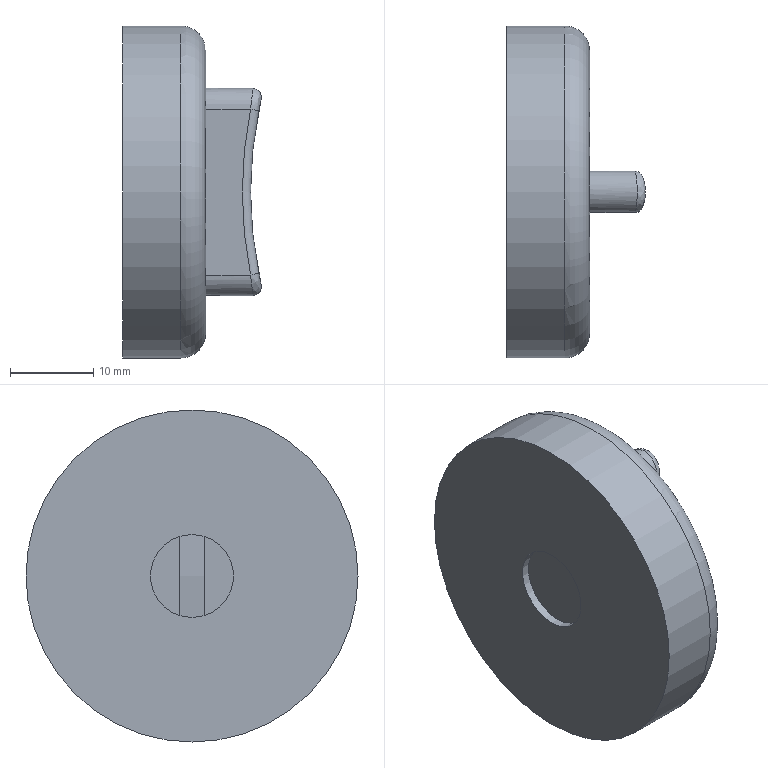Component | NX | KNOB_2 | 1 solid | 23 faces | volume 3582 mm3 | cylinder 9 | plane 8 | torus 4 | spline 2 | commonest cylinder face diameters 3 x2 5 x2 38 x1 102 x1 10 x1 40 x1 100 x1